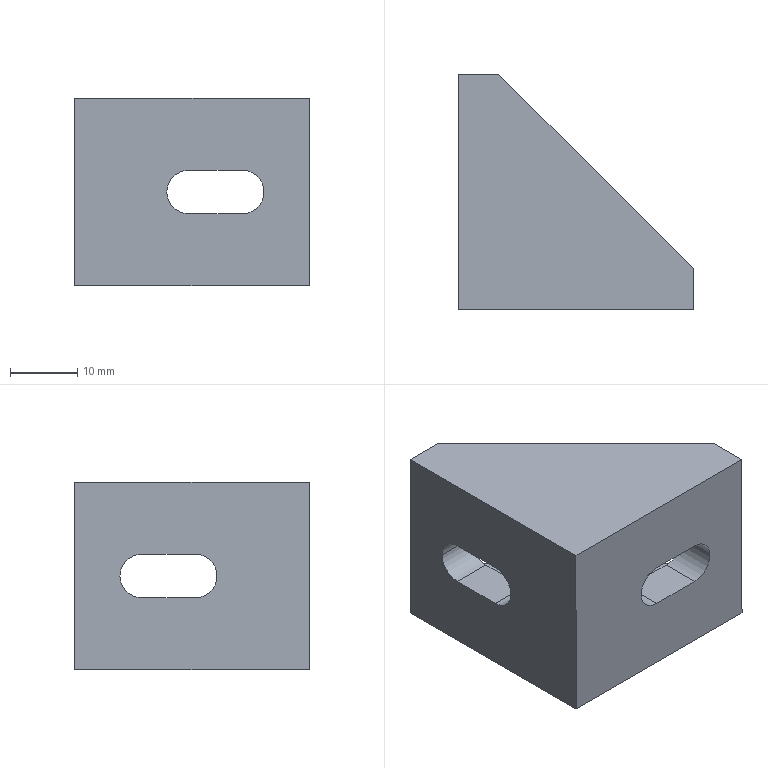Component | SolidWorks | TriangularBracket-6 | 1 solid | 22 faces | box 35 x 35 x 28 mm | volume 14776 mm3 | plane 16 | cylinder 6 | commonest cylinder face diameters 6.5 x6
build123d program:
from build123d import *

# Parameters (mm, degrees)
BOSS_EXTRUDE1_DEPTH = 28
BOSS_EXTRUDE2_DEPTH = 6
BOSS_EXTRUDE3_DEPTH = 6
CUT_EXTRUDE1_DEPTH  = 6
CUT_EXTRUDE2_DEPTH  = 54.385


with BuildPart() as part:
    # Sketch1 → Boss-Extrude1 (new body)
    with BuildSketch(Plane(origin=(0, 0, 0), x_dir=(1, 0, 0), z_dir=(0, 1, 0))):
        Polygon((0, 0), (6, 0), (6, -29), (35, -29), (35, -35), (0, -35), align=None)
    extrude(amount=BOSS_EXTRUDE1_DEPTH)

    # Sketch2 → Boss-Extrude2 (add)
    with BuildSketch(Plane(origin=(0, 28, 0), x_dir=(1, 0, 0), z_dir=(0, 1, 0))):
        Polygon((6, 0), (35, -29), (6, -29), (6, -28.016), align=None)
    extrude(amount=-BOSS_EXTRUDE2_DEPTH)

    # Sketch3 → Boss-Extrude3 (add)
    with BuildSketch(Plane.XZ):
        Polygon((35, 29), (6, 0), (6, 29), align=None)
    extrude(amount=-BOSS_EXTRUDE3_DEPTH)

    # Sketch4 → Cut-Extrude1 (cut)
    with BuildSketch(Plane(origin=(6, 0, 0), x_dir=(0, 0, -1), z_dir=(1, 0, 0))):
        with BuildLine():
            Line((-18, 17.25), (-10, 17.25))
            ThreePointArc((-10, 17.25), (-6.75, 14), (-10, 10.75))
            Line((-10, 10.75), (-18, 10.75))
            ThreePointArc((-18, 10.75), (-21.25, 14), (-18, 17.25))
        make_face()
    extrude(amount=-CUT_EXTRUDE1_DEPTH, mode=Mode.SUBTRACT)

    # Sketch5 → Cut-Extrude2 (cut, through all)
    with BuildSketch(Plane(origin=(0, 0, 29), x_dir=(-1, 0, 0), z_dir=(0, 0, -1))):
        with BuildLine():
            Line((-25, 17.25), (-17, 17.25))
            ThreePointArc((-17, 17.25), (-13.75, 14), (-17, 10.75))
            Line((-17, 10.75), (-25, 10.75))
            ThreePointArc((-25, 10.75), (-28.25, 14), (-25, 17.25))
        make_face()
    extrude(amount=-CUT_EXTRUDE2_DEPTH, mode=Mode.SUBTRACT)


solid = part.part

# Placed as in the assembly
solid = solid.moved(Location((-477.951, 352.323, -325), (90, 0, 0)))
STEP:
#1=COLOUR_RGB('',0.7922,0.8196,0.9333);
#2=FILL_AREA_STYLE_COLOUR('',#1);
#3=FILL_AREA_STYLE('',(#2));
#4=SURFACE_STYLE_FILL_AREA(#3);
#5=SURFACE_SIDE_STYLE('',(#4));
#6=SURFACE_STYLE_USAGE(.BOTH.,#5);
#7=PRESENTATION_STYLE_ASSIGNMENT((#6));
#8=CARTESIAN_POINT('',(-18.276,12.493,-12.244));
#9=VERTEX_POINT('',#8);
#10=CARTESIAN_POINT('',(-18.148,12.493,-12.116));
#11=VERTEX_POINT('',#10);
#12=CARTESIAN_POINT('',(-18.148,12.493,-12.244));
#13=DIRECTION('',(0.,1.,-0.));
#14=DIRECTION('',(-1.,0.,-0.));
#15=AXIS2_PLACEMENT_3D('',#12,#13,#14);
#16=CIRCLE('',#15,0.128);
#17=EDGE_CURVE('',#9,#11,#16,.T.);
#18=ORIENTED_EDGE('',*,*,#17,.F.);
#19=CARTESIAN_POINT('',(-18.276,12.729,-12.244));
#20=VERTEX_POINT('',#19);
#21=CARTESIAN_POINT('',(-18.276,12.493,-12.244));
#22=DIRECTION('',(0.,1.,-0.));
#23=VECTOR('',#22,39.37);
#24=LINE('',#21,#23);
#25=EDGE_CURVE('',#9,#20,#24,.T.);
#26=ORIENTED_EDGE('',*,*,#25,.T.);
#27=CARTESIAN_POINT('',(-18.148,12.729,-12.116));
#28=VERTEX_POINT('',#27);
#29=CARTESIAN_POINT('',(-18.148,12.729,-12.244));
#30=DIRECTION('',(0.,1.,-0.));
#31=DIRECTION('',(-1.,0.,-0.));
#32=AXIS2_PLACEMENT_3D('',#29,#30,#31);
#33=CIRCLE('',#32,0.128);
#34=EDGE_CURVE('',#20,#28,#33,.T.);
#35=ORIENTED_EDGE('',*,*,#34,.T.);
#36=CARTESIAN_POINT('',(-18.148,12.493,-12.116));
#37=DIRECTION('',(0.,1.,-0.));
#38=VECTOR('',#37,39.37);
#39=LINE('',#36,#38);
#40=EDGE_CURVE('',#11,#28,#39,.T.);
#41=ORIENTED_EDGE('',*,*,#40,.F.);
#42=EDGE_LOOP('',(#18,#26,#35,#41));
#43=FACE_OUTER_BOUND('',#42,.T.);
#44=CARTESIAN_POINT('',(-18.148,12.493,-12.244));
#45=DIRECTION('',(0.,1.,-0.));
#46=DIRECTION('',(-1.,0.,-0.));
#47=AXIS2_PLACEMENT_3D('',#44,#45,#46);
#48=CYLINDRICAL_SURFACE('',#47,0.128);
#49=ADVANCED_FACE('',(#43),#48,.F.);
#50=CARTESIAN_POINT('',(-18.817,13.605,-12.244));
#51=VERTEX_POINT('',#50);
#52=CARTESIAN_POINT('',(-18.817,13.477,-12.116));
#53=VERTEX_POINT('',#52);
#54=CARTESIAN_POINT('',(-18.817,13.477,-12.244));
#55=DIRECTION('',(1.,-0.,0.));
#56=DIRECTION('',(0.,1.,0.));
#57=AXIS2_PLACEMENT_3D('',#54,#55,#56);
#58=CIRCLE('',#57,0.128);
#59=EDGE_CURVE('',#51,#53,#58,.T.);
#60=ORIENTED_EDGE('',*,*,#59,.F.);
#61=CARTESIAN_POINT('',(-18.581,13.605,-12.244));
#62=VERTEX_POINT('',#61);
#63=CARTESIAN_POINT('',(-18.817,13.605,-12.244));
#64=DIRECTION('',(1.,-0.,0.));
#65=VECTOR('',#64,39.37);
#66=LINE('',#63,#65);
#67=EDGE_CURVE('',#51,#62,#66,.T.);
#68=ORIENTED_EDGE('',*,*,#67,.T.);
#69=CARTESIAN_POINT('',(-18.581,13.477,-12.116));
#70=VERTEX_POINT('',#69);
#71=CARTESIAN_POINT('',(-18.581,13.477,-12.244));
#72=DIRECTION('',(1.,-0.,0.));
#73=DIRECTION('',(0.,1.,0.));
#74=AXIS2_PLACEMENT_3D('',#71,#72,#73);
#75=CIRCLE('',#74,0.128);
#76=EDGE_CURVE('',#62,#70,#75,.T.);
#77=ORIENTED_EDGE('',*,*,#76,.T.);
#78=CARTESIAN_POINT('',(-18.817,13.477,-12.116));
#79=DIRECTION('',(1.,-0.,0.));
#80=VECTOR('',#79,39.37);
#81=LINE('',#78,#80);
#82=EDGE_CURVE('',#53,#70,#81,.T.);
#83=ORIENTED_EDGE('',*,*,#82,.F.);
#84=EDGE_LOOP('',(#60,#68,#77,#83));
#85=FACE_OUTER_BOUND('',#84,.T.);
#86=CARTESIAN_POINT('',(-18.817,13.477,-12.244));
#87=DIRECTION('',(1.,-0.,0.));
#88=DIRECTION('',(0.,1.,0.));
#89=AXIS2_PLACEMENT_3D('',#86,#87,#88);
#90=CYLINDRICAL_SURFACE('',#89,0.128);
#91=ADVANCED_FACE('',(#85),#90,.F.);
#92=CARTESIAN_POINT('',(-17.833,12.729,-12.372));
#93=VERTEX_POINT('',#92);
#94=CARTESIAN_POINT('',(-18.148,12.729,-12.372));
#95=VERTEX_POINT('',#94);
#96=CARTESIAN_POINT('',(-17.833,12.729,-12.372));
#97=DIRECTION('',(-1.,0.,-0.));
#98=VECTOR('',#97,39.37);
#99=LINE('',#96,#98);
#100=EDGE_CURVE('',#93,#95,#99,.T.);
#101=ORIENTED_EDGE('',*,*,#100,.F.);
#102=CARTESIAN_POINT('',(-17.833,12.729,-12.116));
#103=VERTEX_POINT('',#102);
#104=CARTESIAN_POINT('',(-17.833,12.729,-12.244));
#105=DIRECTION('',(0.,1.,-0.));
#106=DIRECTION('',(-1.,0.,-0.));
#107=AXIS2_PLACEMENT_3D('',#104,#105,#106);
#108=CIRCLE('',#107,0.128);
#109=EDGE_CURVE('',#103,#93,#108,.T.);
#110=ORIENTED_EDGE('',*,*,#109,.F.);
#111=CARTESIAN_POINT('',(-17.833,12.729,-12.116));
#112=DIRECTION('',(1.,-0.,0.));
#113=VECTOR('',#112,39.37);
#114=LINE('',#111,#113);
#115=EDGE_CURVE('',#28,#103,#114,.T.);
#116=ORIENTED_EDGE('',*,*,#115,.F.);
#117=ORIENTED_EDGE('',*,*,#34,.F.);
#118=CARTESIAN_POINT('',(-18.148,12.729,-12.244));
#119=DIRECTION('',(0.,1.,-0.));
#120=DIRECTION('',(-1.,0.,-0.));
#121=AXIS2_PLACEMENT_3D('',#118,#119,#120);
#122=CIRCLE('',#121,0.128);
#123=EDGE_CURVE('',#95,#20,#122,.T.);
#124=ORIENTED_EDGE('',*,*,#123,.F.);
#125=EDGE_LOOP('',(#101,#110,#116,#117,#124));
#126=FACE_BOUND('',#125,.T.);
#127=CARTESIAN_POINT('',(-17.439,12.729,-12.559));
#128=VERTEX_POINT('',#127);
#129=CARTESIAN_POINT('',(-18.581,12.729,-12.559));
#130=VERTEX_POINT('',#129);
#131=CARTESIAN_POINT('',(-18.581,12.729,-12.559));
#132=DIRECTION('',(-1.,0.,-0.));
#133=VECTOR('',#132,39.37);
#134=LINE('',#131,#133);
#135=EDGE_CURVE('',#128,#130,#134,.T.);
#136=ORIENTED_EDGE('',*,*,#135,.T.);
#137=CARTESIAN_POINT('',(-18.581,12.729,-11.929));
#138=VERTEX_POINT('',#137);
#139=CARTESIAN_POINT('',(-18.581,12.729,-11.693));
#140=DIRECTION('',(0.,-0.,-1.));
#141=VECTOR('',#140,39.37);
#142=LINE('',#139,#141);
#143=EDGE_CURVE('',#138,#130,#142,.T.);
#144=ORIENTED_EDGE('',*,*,#143,.F.);
#145=CARTESIAN_POINT('',(-17.439,12.729,-11.929));
#146=VERTEX_POINT('',#145);
#147=CARTESIAN_POINT('',(-17.439,12.729,-11.929));
#148=DIRECTION('',(1.,-0.,0.));
#149=VECTOR('',#148,39.37);
#150=LINE('',#147,#149);
#151=EDGE_CURVE('',#138,#146,#150,.T.);
#152=ORIENTED_EDGE('',*,*,#151,.T.);
#153=CARTESIAN_POINT('',(-17.439,12.729,-11.693));
#154=DIRECTION('',(0.,-0.,-1.));
#155=VECTOR('',#154,39.37);
#156=LINE('',#153,#155);
#157=EDGE_CURVE('',#146,#128,#156,.T.);
#158=ORIENTED_EDGE('',*,*,#157,.T.);
#159=EDGE_LOOP('',(#136,#144,#152,#158));
#160=FACE_OUTER_BOUND('',#159,.T.);
#161=CARTESIAN_POINT('',(-18.581,12.729,-11.693));
#162=DIRECTION('',(-0.,-1.,0.));
#163=DIRECTION('',(1.,-0.,0.));
#164=AXIS2_PLACEMENT_3D('',#161,#162,#163);
#165=PLANE('',#164);
#166=ADVANCED_FACE('',(#126,#160),#165,.F.);
#167=CARTESIAN_POINT('',(-18.581,13.162,-12.372));
#168=VERTEX_POINT('',#167);
#169=CARTESIAN_POINT('',(-18.581,13.477,-12.372));
#170=VERTEX_POINT('',#169);
#171=CARTESIAN_POINT('',(-18.581,13.162,-12.372));
#172=DIRECTION('',(0.,1.,-0.));
#173=VECTOR('',#172,39.37);
#174=LINE('',#171,#173);
#175=EDGE_CURVE('',#168,#170,#174,.T.);
#176=ORIENTED_EDGE('',*,*,#175,.F.);
#177=CARTESIAN_POINT('',(-18.581,13.162,-12.116));
#178=VERTEX_POINT('',#177);
#179=CARTESIAN_POINT('',(-18.581,13.162,-12.244));
#180=DIRECTION('',(1.,-0.,0.));
#181=DIRECTION('',(0.,1.,0.));
#182=AXIS2_PLACEMENT_3D('',#179,#180,#181);
#183=CIRCLE('',#182,0.128);
#184=EDGE_CURVE('',#178,#168,#183,.T.);
#185=ORIENTED_EDGE('',*,*,#184,.F.);
#186=CARTESIAN_POINT('',(-18.581,13.162,-12.116));
#187=DIRECTION('',(-0.,-1.,-0.));
#188=VECTOR('',#187,39.37);
#189=LINE('',#186,#188);
#190=EDGE_CURVE('',#70,#178,#189,.T.);
#191=ORIENTED_EDGE('',*,*,#190,.F.);
#192=ORIENTED_EDGE('',*,*,#76,.F.);
#193=CARTESIAN_POINT('',(-18.581,13.477,-12.244));
#194=DIRECTION('',(1.,-0.,0.));
#195=DIRECTION('',(0.,1.,0.));
#196=AXIS2_PLACEMENT_3D('',#193,#194,#195);
#197=CIRCLE('',#196,0.128);
#198=EDGE_CURVE('',#170,#62,#197,.T.);
#199=ORIENTED_EDGE('',*,*,#198,.F.);
#200=EDGE_LOOP('',(#176,#185,#191,#192,#199));
#201=FACE_BOUND('',#200,.T.);
#202=CARTESIAN_POINT('',(-18.581,13.871,-12.559));
#203=VERTEX_POINT('',#202);
#204=CARTESIAN_POINT('',(-18.581,13.871,-12.559));
#205=DIRECTION('',(0.,1.,-0.));
#206=VECTOR('',#205,39.37);
#207=LINE('',#204,#206);
#208=EDGE_CURVE('',#130,#203,#207,.T.);
#209=ORIENTED_EDGE('',*,*,#208,.T.);
#210=CARTESIAN_POINT('',(-18.581,13.871,-11.929));
#211=VERTEX_POINT('',#210);
#212=CARTESIAN_POINT('',(-18.581,13.871,-11.693));
#213=DIRECTION('',(0.,-0.,-1.));
#214=VECTOR('',#213,39.37);
#215=LINE('',#212,#214);
#216=EDGE_CURVE('',#211,#203,#215,.T.);
#217=ORIENTED_EDGE('',*,*,#216,.F.);
#218=CARTESIAN_POINT('',(-18.581,12.768,-11.929));
#219=DIRECTION('',(-0.,-1.,0.));
#220=VECTOR('',#219,39.37);
#221=LINE('',#218,#220);
#222=EDGE_CURVE('',#211,#138,#221,.T.);
#223=ORIENTED_EDGE('',*,*,#222,.T.);
#224=ORIENTED_EDGE('',*,*,#143,.T.);
#225=EDGE_LOOP('',(#209,#217,#223,#224));
#226=FACE_OUTER_BOUND('',#225,.T.);
#227=CARTESIAN_POINT('',(-18.581,13.871,-11.693));
#228=DIRECTION('',(-1.,0.,-0.));
#229=DIRECTION('',(-0.,-1.,0.));
#230=AXIS2_PLACEMENT_3D('',#227,#228,#229);
#231=PLANE('',#230);
#232=ADVANCED_FACE('',(#201,#226),#231,.F.);
#233=CARTESIAN_POINT('',(-18.817,13.162,-12.116));
#234=VERTEX_POINT('',#233);
#235=CARTESIAN_POINT('',(-18.817,13.162,-12.116));
#236=DIRECTION('',(-0.,-1.,-0.));
#237=VECTOR('',#236,39.37);
#238=LINE('',#235,#237);
#239=EDGE_CURVE('',#53,#234,#238,.T.);
#240=ORIENTED_EDGE('',*,*,#239,.T.);
#241=CARTESIAN_POINT('',(-18.817,13.162,-12.372));
#242=VERTEX_POINT('',#241);
#243=CARTESIAN_POINT('',(-18.817,13.162,-12.244));
#244=DIRECTION('',(1.,-0.,0.));
#245=DIRECTION('',(0.,1.,0.));
#246=AXIS2_PLACEMENT_3D('',#243,#244,#245);
#247=CIRCLE('',#246,0.128);
#248=EDGE_CURVE('',#234,#242,#247,.T.);
#249=ORIENTED_EDGE('',*,*,#248,.T.);
#250=CARTESIAN_POINT('',(-18.817,13.477,-12.372));
#251=VERTEX_POINT('',#250);
#252=CARTESIAN_POINT('',(-18.817,13.162,-12.372));
#253=DIRECTION('',(0.,1.,-0.));
#254=VECTOR('',#253,39.37);
#255=LINE('',#252,#254);
#256=EDGE_CURVE('',#242,#251,#255,.T.);
#257=ORIENTED_EDGE('',*,*,#256,.T.);
#258=CARTESIAN_POINT('',(-18.817,13.477,-12.244));
#259=DIRECTION('',(1.,-0.,0.));
#260=DIRECTION('',(0.,1.,0.));
#261=AXIS2_PLACEMENT_3D('',#258,#259,#260);
#262=CIRCLE('',#261,0.128);
#263=EDGE_CURVE('',#251,#51,#262,.T.);
#264=ORIENTED_EDGE('',*,*,#263,.T.);
#265=ORIENTED_EDGE('',*,*,#59,.T.);
#266=EDGE_LOOP('',(#240,#249,#257,#264,#265));
#267=FACE_BOUND('',#266,.T.);
#268=CARTESIAN_POINT('',(-18.817,13.871,-12.795));
#269=VERTEX_POINT('',#268);
#270=CARTESIAN_POINT('',(-18.817,12.493,-12.795));
#271=VERTEX_POINT('',#270);
#272=CARTESIAN_POINT('',(-18.817,13.871,-12.795));
#273=DIRECTION('',(-0.,-1.,0.));
#274=VECTOR('',#273,39.37);
#275=LINE('',#272,#274);
#276=EDGE_CURVE('',#269,#271,#275,.T.);
#277=ORIENTED_EDGE('',*,*,#276,.T.);
#278=CARTESIAN_POINT('',(-18.817,12.493,-11.693));
#279=VERTEX_POINT('',#278);
#280=CARTESIAN_POINT('',(-18.817,12.493,-11.693));
#281=DIRECTION('',(0.,-0.,-1.));
#282=VECTOR('',#281,39.37);
#283=LINE('',#280,#282);
#284=EDGE_CURVE('',#279,#271,#283,.T.);
#285=ORIENTED_EDGE('',*,*,#284,.F.);
#286=CARTESIAN_POINT('',(-18.817,13.871,-11.693));
#287=VERTEX_POINT('',#286);
#288=CARTESIAN_POINT('',(-18.817,13.871,-11.693));
#289=DIRECTION('',(-0.,-1.,0.));
#290=VECTOR('',#289,39.37);
#291=LINE('',#288,#290);
#292=EDGE_CURVE('',#287,#279,#291,.T.);
#293=ORIENTED_EDGE('',*,*,#292,.F.);
#294=CARTESIAN_POINT('',(-18.817,13.871,-11.693));
#295=DIRECTION('',(0.,-0.,-1.));
#296=VECTOR('',#295,39.37);
#297=LINE('',#294,#296);
#298=EDGE_CURVE('',#287,#269,#297,.T.);
#299=ORIENTED_EDGE('',*,*,#298,.T.);
#300=EDGE_LOOP('',(#277,#285,#293,#299));
#301=FACE_OUTER_BOUND('',#300,.T.);
#302=CARTESIAN_POINT('',(-18.817,13.871,-11.693));
#303=DIRECTION('',(1.,-0.,0.));
#304=DIRECTION('',(0.,1.,-0.));
#305=AXIS2_PLACEMENT_3D('',#302,#303,#304);
#306=PLANE('',#305);
#307=ADVANCED_FACE('',(#267,#301),#306,.F.);
#308=CARTESIAN_POINT('',(-17.833,12.493,-12.116));
#309=VERTEX_POINT('',#308);
#310=CARTESIAN_POINT('',(-17.833,12.493,-12.116));
#311=DIRECTION('',(1.,-0.,0.));
#312=VECTOR('',#311,39.37);
#313=LINE('',#310,#312);
#314=EDGE_CURVE('',#11,#309,#313,.T.);
#315=ORIENTED_EDGE('',*,*,#314,.T.);
#316=CARTESIAN_POINT('',(-17.833,12.493,-12.372));
#317=VERTEX_POINT('',#316);
#318=CARTESIAN_POINT('',(-17.833,12.493,-12.244));
#319=DIRECTION('',(0.,1.,-0.));
#320=DIRECTION('',(-1.,0.,-0.));
#321=AXIS2_PLACEMENT_3D('',#318,#319,#320);
#322=CIRCLE('',#321,0.128);
#323=EDGE_CURVE('',#309,#317,#322,.T.);
#324=ORIENTED_EDGE('',*,*,#323,.T.);
#325=CARTESIAN_POINT('',(-18.148,12.493,-12.372));
#326=VERTEX_POINT('',#325);
#327=CARTESIAN_POINT('',(-17.833,12.493,-12.372));
#328=DIRECTION('',(-1.,0.,-0.));
#329=VECTOR('',#328,39.37);
#330=LINE('',#327,#329);
#331=EDGE_CURVE('',#317,#326,#330,.T.);
#332=ORIENTED_EDGE('',*,*,#331,.T.);
#333=CARTESIAN_POINT('',(-18.148,12.493,-12.244));
#334=DIRECTION('',(0.,1.,-0.));
#335=DIRECTION('',(-1.,0.,-0.));
#336=AXIS2_PLACEMENT_3D('',#333,#334,#335);
#337=CIRCLE('',#336,0.128);
#338=EDGE_CURVE('',#326,#9,#337,.T.);
#339=ORIENTED_EDGE('',*,*,#338,.T.);
#340=ORIENTED_EDGE('',*,*,#17,.T.);
#341=EDGE_LOOP('',(#315,#324,#332,#339,#340));
#342=FACE_BOUND('',#341,.T.);
#343=CARTESIAN_POINT('',(-17.439,12.493,-12.795));
#344=VERTEX_POINT('',#343);
#345=CARTESIAN_POINT('',(-18.817,12.493,-12.795));
#346=DIRECTION('',(1.,-0.,0.));
#347=VECTOR('',#346,39.37);
#348=LINE('',#345,#347);
#349=EDGE_CURVE('',#271,#344,#348,.T.);
#350=ORIENTED_EDGE('',*,*,#349,.T.);
#351=CARTESIAN_POINT('',(-17.439,12.493,-11.693));
#352=VERTEX_POINT('',#351);
#353=CARTESIAN_POINT('',(-17.439,12.493,-11.693));
#354=DIRECTION('',(0.,-0.,-1.));
#355=VECTOR('',#354,39.37);
#356=LINE('',#353,#355);
#357=EDGE_CURVE('',#352,#344,#356,.T.);
#358=ORIENTED_EDGE('',*,*,#357,.F.);
#359=CARTESIAN_POINT('',(-18.817,12.493,-11.693));
#360=DIRECTION('',(1.,-0.,0.));
#361=VECTOR('',#360,39.37);
#362=LINE('',#359,#361);
#363=EDGE_CURVE('',#279,#352,#362,.T.);
#364=ORIENTED_EDGE('',*,*,#363,.F.);
#365=ORIENTED_EDGE('',*,*,#284,.T.);
#366=EDGE_LOOP('',(#350,#358,#364,#365));
#367=FACE_OUTER_BOUND('',#366,.T.);
#368=CARTESIAN_POINT('',(-18.817,12.493,-11.693));
#369=DIRECTION('',(0.,1.,-0.));
#370=DIRECTION('',(-1.,0.,-0.));
#371=AXIS2_PLACEMENT_3D('',#368,#369,#370);
#372=PLANE('',#371);
#373=ADVANCED_FACE('',(#342,#367),#372,.F.);
#374=CARTESIAN_POINT('',(-17.439,12.729,-12.795));
#375=VERTEX_POINT('',#374);
#376=CARTESIAN_POINT('',(-17.439,12.729,-12.795));
#377=DIRECTION('',(-0.,1.,-0.));
#378=VECTOR('',#377,39.37);
#379=LINE('',#376,#378);
#380=EDGE_CURVE('',#344,#375,#379,.T.);
#381=ORIENTED_EDGE('',*,*,#380,.T.);
#382=CARTESIAN_POINT('',(-17.439,12.729,-12.559));
#383=DIRECTION('',(0.,-0.,-1.));
#384=VECTOR('',#383,39.37);
#385=LINE('',#382,#384);
#386=EDGE_CURVE('',#128,#375,#385,.T.);
#387=ORIENTED_EDGE('',*,*,#386,.F.);
#388=ORIENTED_EDGE('',*,*,#157,.F.);
#389=CARTESIAN_POINT('',(-17.439,12.729,-11.693));
#390=VERTEX_POINT('',#389);
#391=CARTESIAN_POINT('',(-17.439,12.729,-11.693));
#392=DIRECTION('',(0.,-0.,-1.));
#393=VECTOR('',#392,39.37);
#394=LINE('',#391,#393);
#395=EDGE_CURVE('',#390,#146,#394,.T.);
#396=ORIENTED_EDGE('',*,*,#395,.F.);
#397=CARTESIAN_POINT('',(-17.439,12.729,-11.693));
#398=DIRECTION('',(-0.,1.,-0.));
#399=VECTOR('',#398,39.37);
#400=LINE('',#397,#399);
#401=EDGE_CURVE('',#352,#390,#400,.T.);
#402=ORIENTED_EDGE('',*,*,#401,.F.);
#403=ORIENTED_EDGE('',*,*,#357,.T.);
#404=EDGE_LOOP('',(#381,#387,#388,#396,#402,#403));
#405=FACE_OUTER_BOUND('',#404,.T.);
#406=CARTESIAN_POINT('',(-17.439,12.729,-11.693));
#407=DIRECTION('',(-1.,-0.,-0.));
#408=DIRECTION('',(0.,-1.,0.));
#409=AXIS2_PLACEMENT_3D('',#406,#407,#408);
#410=PLANE('',#409);
#411=ADVANCED_FACE('',(#405),#410,.F.);
#412=CARTESIAN_POINT('',(-18.581,13.871,-12.795));
#413=VERTEX_POINT('',#412);
#414=CARTESIAN_POINT('',(-18.817,13.871,-12.795));
#415=DIRECTION('',(-1.,0.,-0.));
#416=VECTOR('',#415,39.37);
#417=LINE('',#414,#416);
#418=EDGE_CURVE('',#413,#269,#417,.T.);
#419=ORIENTED_EDGE('',*,*,#418,.T.);
#420=ORIENTED_EDGE('',*,*,#298,.F.);
#421=CARTESIAN_POINT('',(-18.581,13.871,-11.693));
#422=VERTEX_POINT('',#421);
#423=CARTESIAN_POINT('',(-18.817,13.871,-11.693));
#424=DIRECTION('',(-1.,0.,-0.));
#425=VECTOR('',#424,39.37);
#426=LINE('',#423,#425);
#427=EDGE_CURVE('',#422,#287,#426,.T.);
#428=ORIENTED_EDGE('',*,*,#427,.F.);
#429=CARTESIAN_POINT('',(-18.581,13.871,-11.693));
#430=DIRECTION('',(0.,-0.,-1.));
#431=VECTOR('',#430,39.37);
#432=LINE('',#429,#431);
#433=EDGE_CURVE('',#422,#211,#432,.T.);
#434=ORIENTED_EDGE('',*,*,#433,.T.);
#435=ORIENTED_EDGE('',*,*,#216,.T.);
#436=CARTESIAN_POINT('',(-18.581,13.871,-12.559));
#437=DIRECTION('',(0.,-0.,-1.));
#438=VECTOR('',#437,39.37);
#439=LINE('',#436,#438);
#440=EDGE_CURVE('',#203,#413,#439,.T.);
#441=ORIENTED_EDGE('',*,*,#440,.T.);
#442=EDGE_LOOP('',(#419,#420,#428,#434,#435,#441));
#443=FACE_OUTER_BOUND('',#442,.T.);
#444=CARTESIAN_POINT('',(-18.817,13.871,-11.693));
#445=DIRECTION('',(-0.,-1.,0.));
#446=DIRECTION('',(1.,-0.,0.));
#447=AXIS2_PLACEMENT_3D('',#444,#445,#446);
#448=PLANE('',#447);
#449=ADVANCED_FACE('',(#443),#448,.F.);
#450=ORIENTED_EDGE('',*,*,#292,.T.);
#451=ORIENTED_EDGE('',*,*,#363,.T.);
#452=ORIENTED_EDGE('',*,*,#401,.T.);
#453=CARTESIAN_POINT('',(-18.581,13.871,-11.693));
#454=DIRECTION('',(-0.7071,0.7071,-0.));
#455=VECTOR('',#454,39.37);
#456=LINE('',#453,#455);
#457=EDGE_CURVE('',#390,#422,#456,.T.);
#458=ORIENTED_EDGE('',*,*,#457,.T.);
#459=ORIENTED_EDGE('',*,*,#427,.T.);
#460=EDGE_LOOP('',(#450,#451,#452,#458,#459));
#461=FACE_OUTER_BOUND('',#460,.T.);
#462=CARTESIAN_POINT('',(-18.817,13.871,-11.693));
#463=DIRECTION('',(-0.,0.,1.));
#464=DIRECTION('',(-0.,-1.,0.));
#465=AXIS2_PLACEMENT_3D('',#462,#463,#464);
#466=PLANE('',#465);
#467=ADVANCED_FACE('',(#461),#466,.T.);
#468=ORIENTED_EDGE('',*,*,#276,.F.);
#469=ORIENTED_EDGE('',*,*,#418,.F.);
#470=CARTESIAN_POINT('',(-17.439,12.729,-12.795));
#471=DIRECTION('',(0.7071,-0.7071,0.));
#472=VECTOR('',#471,39.37);
#473=LINE('',#470,#472);
#474=EDGE_CURVE('',#413,#375,#473,.T.);
#475=ORIENTED_EDGE('',*,*,#474,.T.);
#476=ORIENTED_EDGE('',*,*,#380,.F.);
#477=ORIENTED_EDGE('',*,*,#349,.F.);
#478=EDGE_LOOP('',(#468,#469,#475,#476,#477));
#479=FACE_OUTER_BOUND('',#478,.T.);
#480=CARTESIAN_POINT('',(-18.817,13.871,-12.795));
#481=DIRECTION('',(-0.,0.,1.));
#482=DIRECTION('',(-0.,-1.,0.));
#483=AXIS2_PLACEMENT_3D('',#480,#481,#482);
#484=PLANE('',#483);
#485=ADVANCED_FACE('',(#479),#484,.F.);
#486=ORIENTED_EDGE('',*,*,#457,.F.);
#487=ORIENTED_EDGE('',*,*,#395,.T.);
#488=CARTESIAN_POINT('',(-18.581,13.871,-11.929));
#489=DIRECTION('',(-0.7071,0.7071,-0.));
#490=VECTOR('',#489,39.37);
#491=LINE('',#488,#490);
#492=EDGE_CURVE('',#146,#211,#491,.T.);
#493=ORIENTED_EDGE('',*,*,#492,.T.);
#494=ORIENTED_EDGE('',*,*,#433,.F.);
#495=EDGE_LOOP('',(#486,#487,#493,#494));
#496=FACE_OUTER_BOUND('',#495,.T.);
#497=CARTESIAN_POINT('',(-18.581,13.871,-11.929));
#498=DIRECTION('',(0.7071,0.7071,0.));
#499=DIRECTION('',(-0.7071,0.7071,-0.));
#500=AXIS2_PLACEMENT_3D('',#497,#498,#499);
#501=PLANE('',#500);
#502=ADVANCED_FACE('',(#496),#501,.T.);
#503=ORIENTED_EDGE('',*,*,#222,.F.);
#504=ORIENTED_EDGE('',*,*,#492,.F.);
#505=ORIENTED_EDGE('',*,*,#151,.F.);
#506=EDGE_LOOP('',(#503,#504,#505));
#507=FACE_OUTER_BOUND('',#506,.T.);
#508=CARTESIAN_POINT('',(-18.817,13.871,-11.929));
#509=DIRECTION('',(-0.,0.,1.));
#510=DIRECTION('',(-0.,-1.,0.));
#511=AXIS2_PLACEMENT_3D('',#508,#509,#510);
#512=PLANE('',#511);
#513=ADVANCED_FACE('',(#507),#512,.F.);
#514=ORIENTED_EDGE('',*,*,#474,.F.);
#515=ORIENTED_EDGE('',*,*,#440,.F.);
#516=CARTESIAN_POINT('',(-17.439,12.729,-12.559));
#517=DIRECTION('',(0.7071,-0.7071,0.));
#518=VECTOR('',#517,39.37);
#519=LINE('',#516,#518);
#520=EDGE_CURVE('',#203,#128,#519,.T.);
#521=ORIENTED_EDGE('',*,*,#520,.T.);
#522=ORIENTED_EDGE('',*,*,#386,.T.);
#523=EDGE_LOOP('',(#514,#515,#521,#522));
#524=FACE_OUTER_BOUND('',#523,.T.);
#525=CARTESIAN_POINT('',(-17.439,12.729,-12.559));
#526=DIRECTION('',(0.7071,0.7071,0.));
#527=DIRECTION('',(-0.7071,0.7071,-0.));
#528=AXIS2_PLACEMENT_3D('',#525,#526,#527);
#529=PLANE('',#528);
#530=ADVANCED_FACE('',(#524),#529,.T.);
#531=ORIENTED_EDGE('',*,*,#135,.F.);
#532=ORIENTED_EDGE('',*,*,#520,.F.);
#533=ORIENTED_EDGE('',*,*,#208,.F.);
#534=EDGE_LOOP('',(#531,#532,#533));
#535=FACE_OUTER_BOUND('',#534,.T.);
#536=CARTESIAN_POINT('',(-18.817,13.871,-12.559));
#537=DIRECTION('',(0.,-0.,-1.));
#538=DIRECTION('',(0.,1.,-0.));
#539=AXIS2_PLACEMENT_3D('',#536,#537,#538);
#540=PLANE('',#539);
#541=ADVANCED_FACE('',(#535),#540,.F.);
#542=ORIENTED_EDGE('',*,*,#184,.T.);
#543=CARTESIAN_POINT('',(-18.817,13.162,-12.372));
#544=DIRECTION('',(1.,-0.,0.));
#545=VECTOR('',#544,39.37);
#546=LINE('',#543,#545);
#547=EDGE_CURVE('',#242,#168,#546,.T.);
#548=ORIENTED_EDGE('',*,*,#547,.F.);
#549=ORIENTED_EDGE('',*,*,#248,.F.);
#550=CARTESIAN_POINT('',(-18.817,13.162,-12.116));
#551=DIRECTION('',(1.,-0.,0.));
#552=VECTOR('',#551,39.37);
#553=LINE('',#550,#552);
#554=EDGE_CURVE('',#234,#178,#553,.T.);
#555=ORIENTED_EDGE('',*,*,#554,.T.);
#556=EDGE_LOOP('',(#542,#548,#549,#555));
#557=FACE_OUTER_BOUND('',#556,.T.);
#558=CARTESIAN_POINT('',(-18.817,13.162,-12.244));
#559=DIRECTION('',(1.,-0.,0.));
#560=DIRECTION('',(0.,1.,0.));
#561=AXIS2_PLACEMENT_3D('',#558,#559,#560);
#562=CYLINDRICAL_SURFACE('',#561,0.128);
#563=ADVANCED_FACE('',(#557),#562,.F.);
#564=ORIENTED_EDGE('',*,*,#190,.T.);
#565=ORIENTED_EDGE('',*,*,#554,.F.);
#566=ORIENTED_EDGE('',*,*,#239,.F.);
#567=ORIENTED_EDGE('',*,*,#82,.T.);
#568=EDGE_LOOP('',(#564,#565,#566,#567));
#569=FACE_OUTER_BOUND('',#568,.T.);
#570=CARTESIAN_POINT('',(-18.817,13.162,-12.116));
#571=DIRECTION('',(-0.,-0.,1.));
#572=DIRECTION('',(-0.,-1.,-0.));
#573=AXIS2_PLACEMENT_3D('',#570,#571,#572);
#574=PLANE('',#573);
#575=ADVANCED_FACE('',(#569),#574,.F.);
#576=ORIENTED_EDGE('',*,*,#67,.F.);
#577=ORIENTED_EDGE('',*,*,#263,.F.);
#578=CARTESIAN_POINT('',(-18.817,13.477,-12.372));
#579=DIRECTION('',(1.,-0.,0.));
#580=VECTOR('',#579,39.37);
#581=LINE('',#578,#580);
#582=EDGE_CURVE('',#251,#170,#581,.T.);
#583=ORIENTED_EDGE('',*,*,#582,.T.);
#584=ORIENTED_EDGE('',*,*,#198,.T.);
#585=EDGE_LOOP('',(#576,#577,#583,#584));
#586=FACE_OUTER_BOUND('',#585,.T.);
#587=CARTESIAN_POINT('',(-18.817,13.477,-12.244));
#588=DIRECTION('',(1.,-0.,0.));
#589=DIRECTION('',(0.,1.,0.));
#590=AXIS2_PLACEMENT_3D('',#587,#588,#589);
#591=CYLINDRICAL_SURFACE('',#590,0.128);
#592=ADVANCED_FACE('',(#586),#591,.F.);
#593=ORIENTED_EDGE('',*,*,#175,.T.);
#594=ORIENTED_EDGE('',*,*,#582,.F.);
#595=ORIENTED_EDGE('',*,*,#256,.F.);
#596=ORIENTED_EDGE('',*,*,#547,.T.);
#597=EDGE_LOOP('',(#593,#594,#595,#596));
#598=FACE_OUTER_BOUND('',#597,.T.);
#599=CARTESIAN_POINT('',(-18.817,13.162,-12.372));
#600=DIRECTION('',(0.,-0.,-1.));
#601=DIRECTION('',(0.,1.,-0.));
#602=AXIS2_PLACEMENT_3D('',#599,#600,#601);
#603=PLANE('',#602);
#604=ADVANCED_FACE('',(#598),#603,.F.);
#605=ORIENTED_EDGE('',*,*,#109,.T.);
#606=CARTESIAN_POINT('',(-17.833,12.493,-12.372));
#607=DIRECTION('',(0.,1.,-0.));
#608=VECTOR('',#607,39.37);
#609=LINE('',#606,#608);
#610=EDGE_CURVE('',#317,#93,#609,.T.);
#611=ORIENTED_EDGE('',*,*,#610,.F.);
#612=ORIENTED_EDGE('',*,*,#323,.F.);
#613=CARTESIAN_POINT('',(-17.833,12.493,-12.116));
#614=DIRECTION('',(0.,1.,-0.));
#615=VECTOR('',#614,39.37);
#616=LINE('',#613,#615);
#617=EDGE_CURVE('',#309,#103,#616,.T.);
#618=ORIENTED_EDGE('',*,*,#617,.T.);
#619=EDGE_LOOP('',(#605,#611,#612,#618));
#620=FACE_OUTER_BOUND('',#619,.T.);
#621=CARTESIAN_POINT('',(-17.833,12.493,-12.244));
#622=DIRECTION('',(0.,1.,-0.));
#623=DIRECTION('',(-1.,0.,-0.));
#624=AXIS2_PLACEMENT_3D('',#621,#622,#623);
#625=CYLINDRICAL_SURFACE('',#624,0.128);
#626=ADVANCED_FACE('',(#620),#625,.F.);
#627=ORIENTED_EDGE('',*,*,#115,.T.);
#628=ORIENTED_EDGE('',*,*,#617,.F.);
#629=ORIENTED_EDGE('',*,*,#314,.F.);
#630=ORIENTED_EDGE('',*,*,#40,.T.);
#631=EDGE_LOOP('',(#627,#628,#629,#630));
#632=FACE_OUTER_BOUND('',#631,.T.);
#633=CARTESIAN_POINT('',(-17.833,12.493,-12.116));
#634=DIRECTION('',(-0.,0.,1.));
#635=DIRECTION('',(-0.,-1.,0.));
#636=AXIS2_PLACEMENT_3D('',#633,#634,#635);
#637=PLANE('',#636);
#638=ADVANCED_FACE('',(#632),#637,.F.);
#639=ORIENTED_EDGE('',*,*,#25,.F.);
#640=ORIENTED_EDGE('',*,*,#338,.F.);
#641=CARTESIAN_POINT('',(-18.148,12.493,-12.372));
#642=DIRECTION('',(0.,1.,-0.));
#643=VECTOR('',#642,39.37);
#644=LINE('',#641,#643);
#645=EDGE_CURVE('',#326,#95,#644,.T.);
#646=ORIENTED_EDGE('',*,*,#645,.T.);
#647=ORIENTED_EDGE('',*,*,#123,.T.);
#648=EDGE_LOOP('',(#639,#640,#646,#647));
#649=FACE_OUTER_BOUND('',#648,.T.);
#650=CARTESIAN_POINT('',(-18.148,12.493,-12.244));
#651=DIRECTION('',(0.,1.,-0.));
#652=DIRECTION('',(-1.,0.,-0.));
#653=AXIS2_PLACEMENT_3D('',#650,#651,#652);
#654=CYLINDRICAL_SURFACE('',#653,0.128);
#655=ADVANCED_FACE('',(#649),#654,.F.);
#656=ORIENTED_EDGE('',*,*,#100,.T.);
#657=ORIENTED_EDGE('',*,*,#645,.F.);
#658=ORIENTED_EDGE('',*,*,#331,.F.);
#659=ORIENTED_EDGE('',*,*,#610,.T.);
#660=EDGE_LOOP('',(#656,#657,#658,#659));
#661=FACE_OUTER_BOUND('',#660,.T.);
#662=CARTESIAN_POINT('',(-17.833,12.493,-12.372));
#663=DIRECTION('',(0.,-0.,-1.));
#664=DIRECTION('',(0.,1.,-0.));
#665=AXIS2_PLACEMENT_3D('',#662,#663,#664);
#666=PLANE('',#665);
#667=ADVANCED_FACE('',(#661),#666,.F.);
#668=CLOSED_SHELL('',(#49,#91,#166,#232,#307,#373,#411,#449,#467,#485,#502,#513,#530,#541,#563,#575,#592,#604,#626,#638,#655,#667));
#669=MANIFOLD_SOLID_BREP('',#668);
#670=STYLED_ITEM('',(#7),#669);
#671=PRESENTATION_LAYER_ASSIGNMENT('','',(#670));
#672=(LENGTH_UNIT()NAMED_UNIT(*)SI_UNIT($,.METRE.));
#673=LENGTH_MEASURE_WITH_UNIT(LENGTH_MEASURE(0.0254),#672);
#674=DIMENSIONAL_EXPONENTS(1.,0.,0.,0.,0.,0.,0.);
#675=(CONVERSION_BASED_UNIT('',#673)LENGTH_UNIT()NAMED_UNIT(#674));
#676=UNCERTAINTY_MEASURE_WITH_UNIT(LENGTH_MEASURE(0.00001),#675,'','');
#677=(NAMED_UNIT(*)PLANE_ANGLE_UNIT()SI_UNIT($,.RADIAN.));
#678=(NAMED_UNIT(*)SI_UNIT($,.STERADIAN.)SOLID_ANGLE_UNIT());
#679=(GEOMETRIC_REPRESENTATION_CONTEXT(3)GLOBAL_UNCERTAINTY_ASSIGNED_CONTEXT((#676))GLOBAL_UNIT_ASSIGNED_CONTEXT((#675,#677,#678))REPRESENTATION_CONTEXT('',''));
#680=MECHANICAL_DESIGN_GEOMETRIC_PRESENTATION_REPRESENTATION('',(#670),#679);
#681=CARTESIAN_POINT('',(0.,0.,0.));
#682=DIRECTION('',(0.,0.,1.));
#683=DIRECTION('',(1.,0.,0.));
#684=AXIS2_PLACEMENT_3D('',#681,#682,#683);
#685=(LENGTH_UNIT()NAMED_UNIT(*)SI_UNIT($,.METRE.));
#686=LENGTH_MEASURE_WITH_UNIT(LENGTH_MEASURE(0.0254),#685);
#687=DIMENSIONAL_EXPONENTS(1.,0.,0.,0.,0.,0.,0.);
#688=(CONVERSION_BASED_UNIT('',#686)LENGTH_UNIT()NAMED_UNIT(#687));
#689=UNCERTAINTY_MEASURE_WITH_UNIT(LENGTH_MEASURE(0.00001),#688,'','');
#690=(NAMED_UNIT(*)PLANE_ANGLE_UNIT()SI_UNIT($,.RADIAN.));
#691=(NAMED_UNIT(*)SI_UNIT($,.STERADIAN.)SOLID_ANGLE_UNIT());
#692=(GEOMETRIC_REPRESENTATION_CONTEXT(3)GLOBAL_UNCERTAINTY_ASSIGNED_CONTEXT((#689))GLOBAL_UNIT_ASSIGNED_CONTEXT((#688,#690,#691))REPRESENTATION_CONTEXT('',''));
#693=ADVANCED_BREP_SHAPE_REPRESENTATION('',(#669,#684),#692);